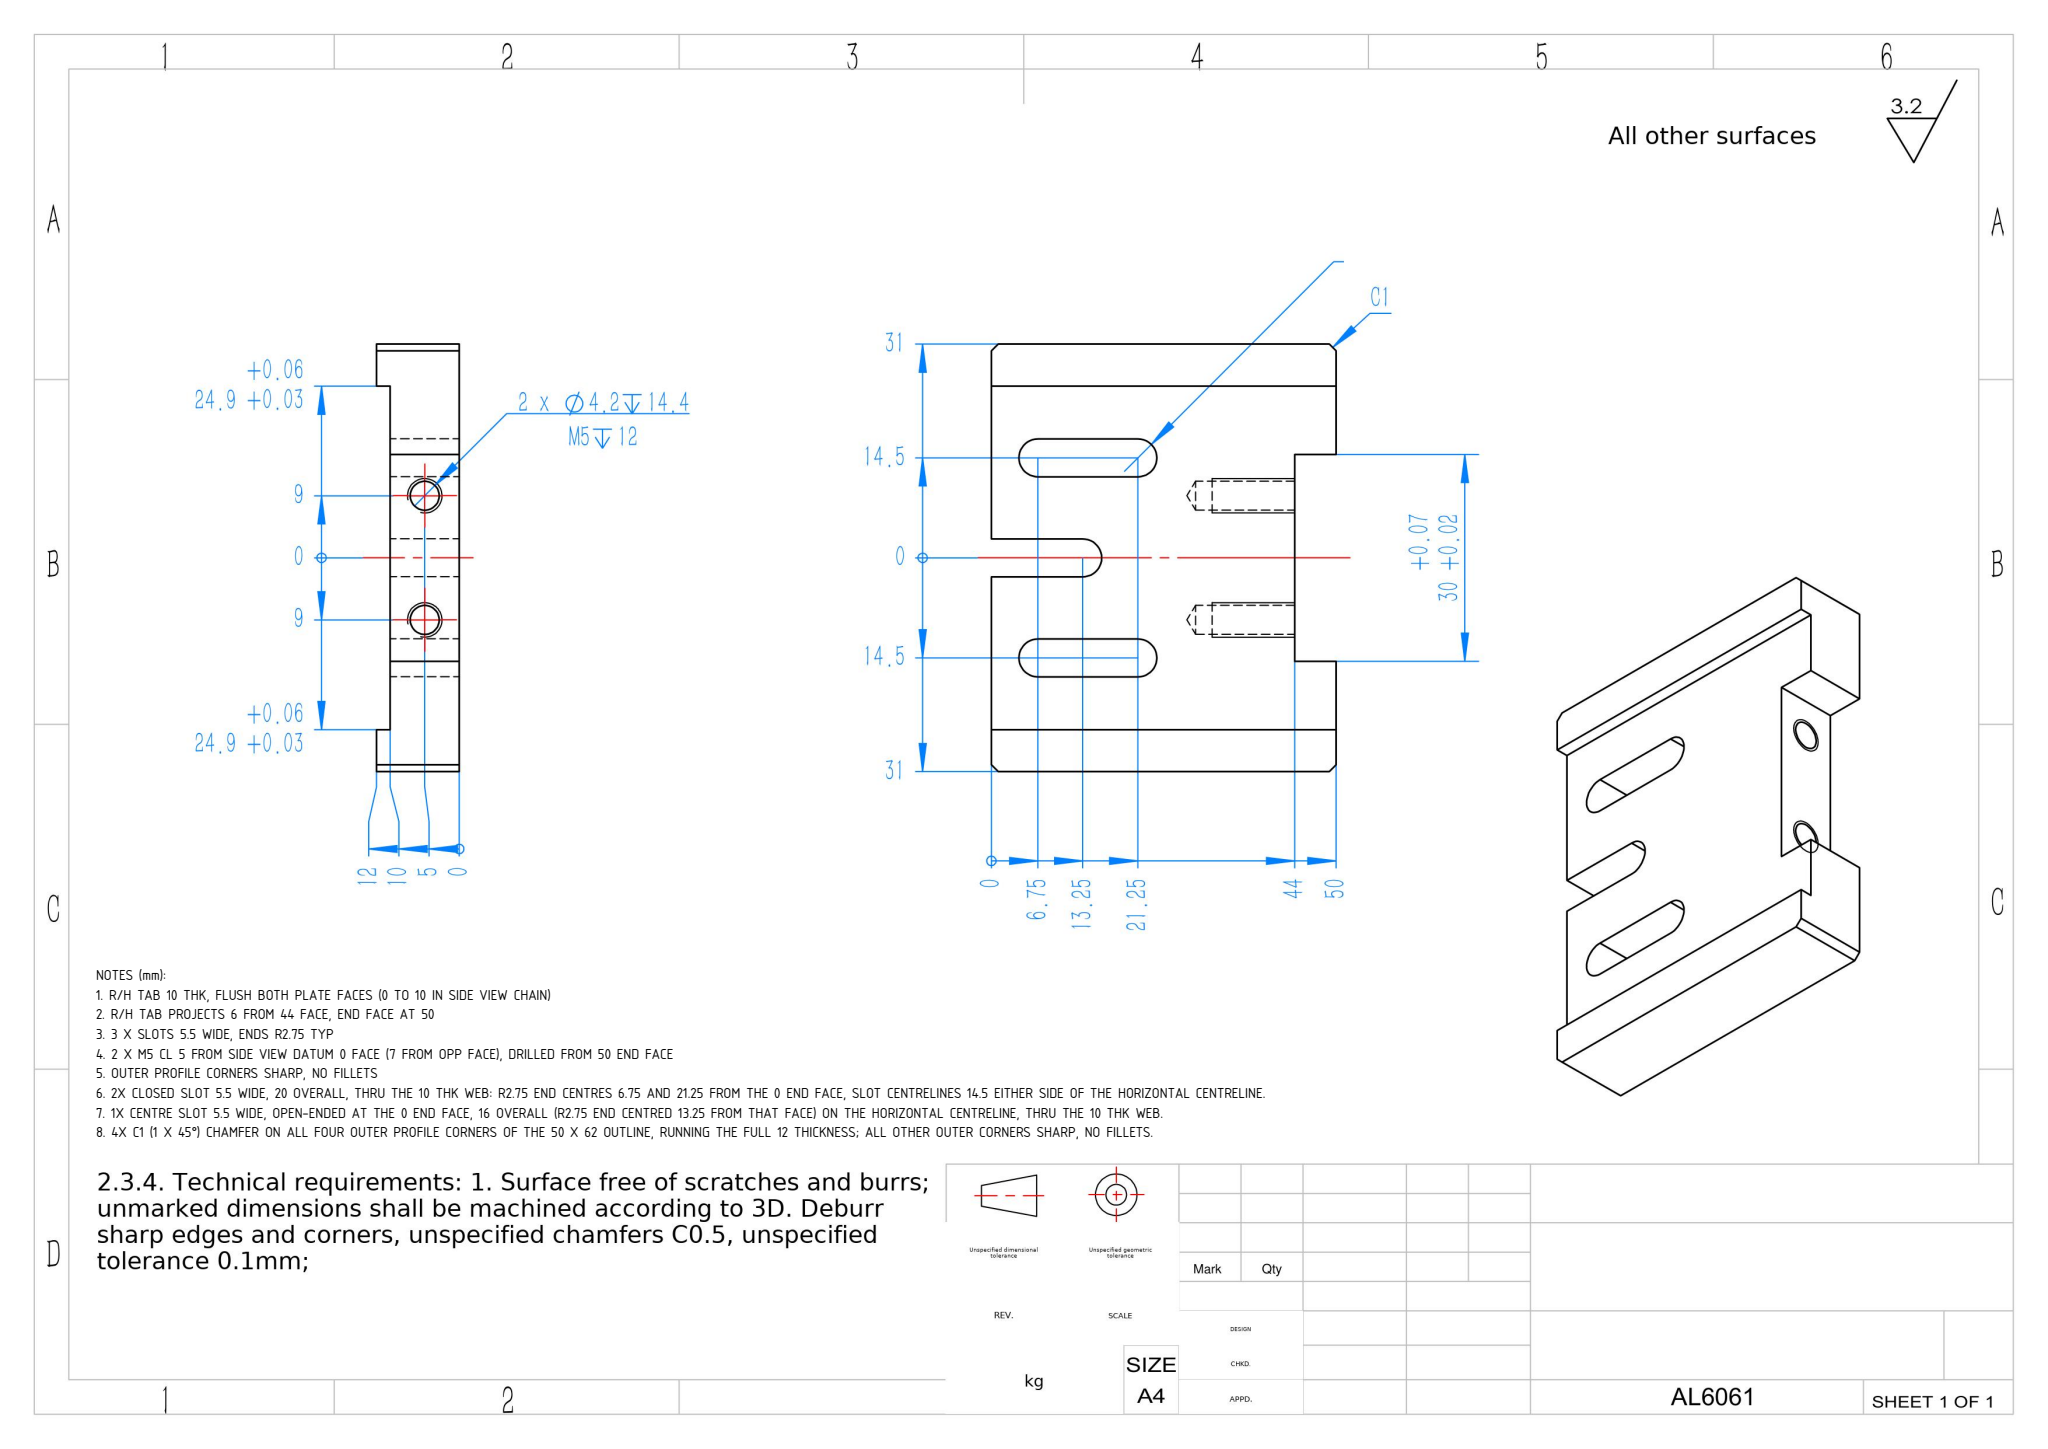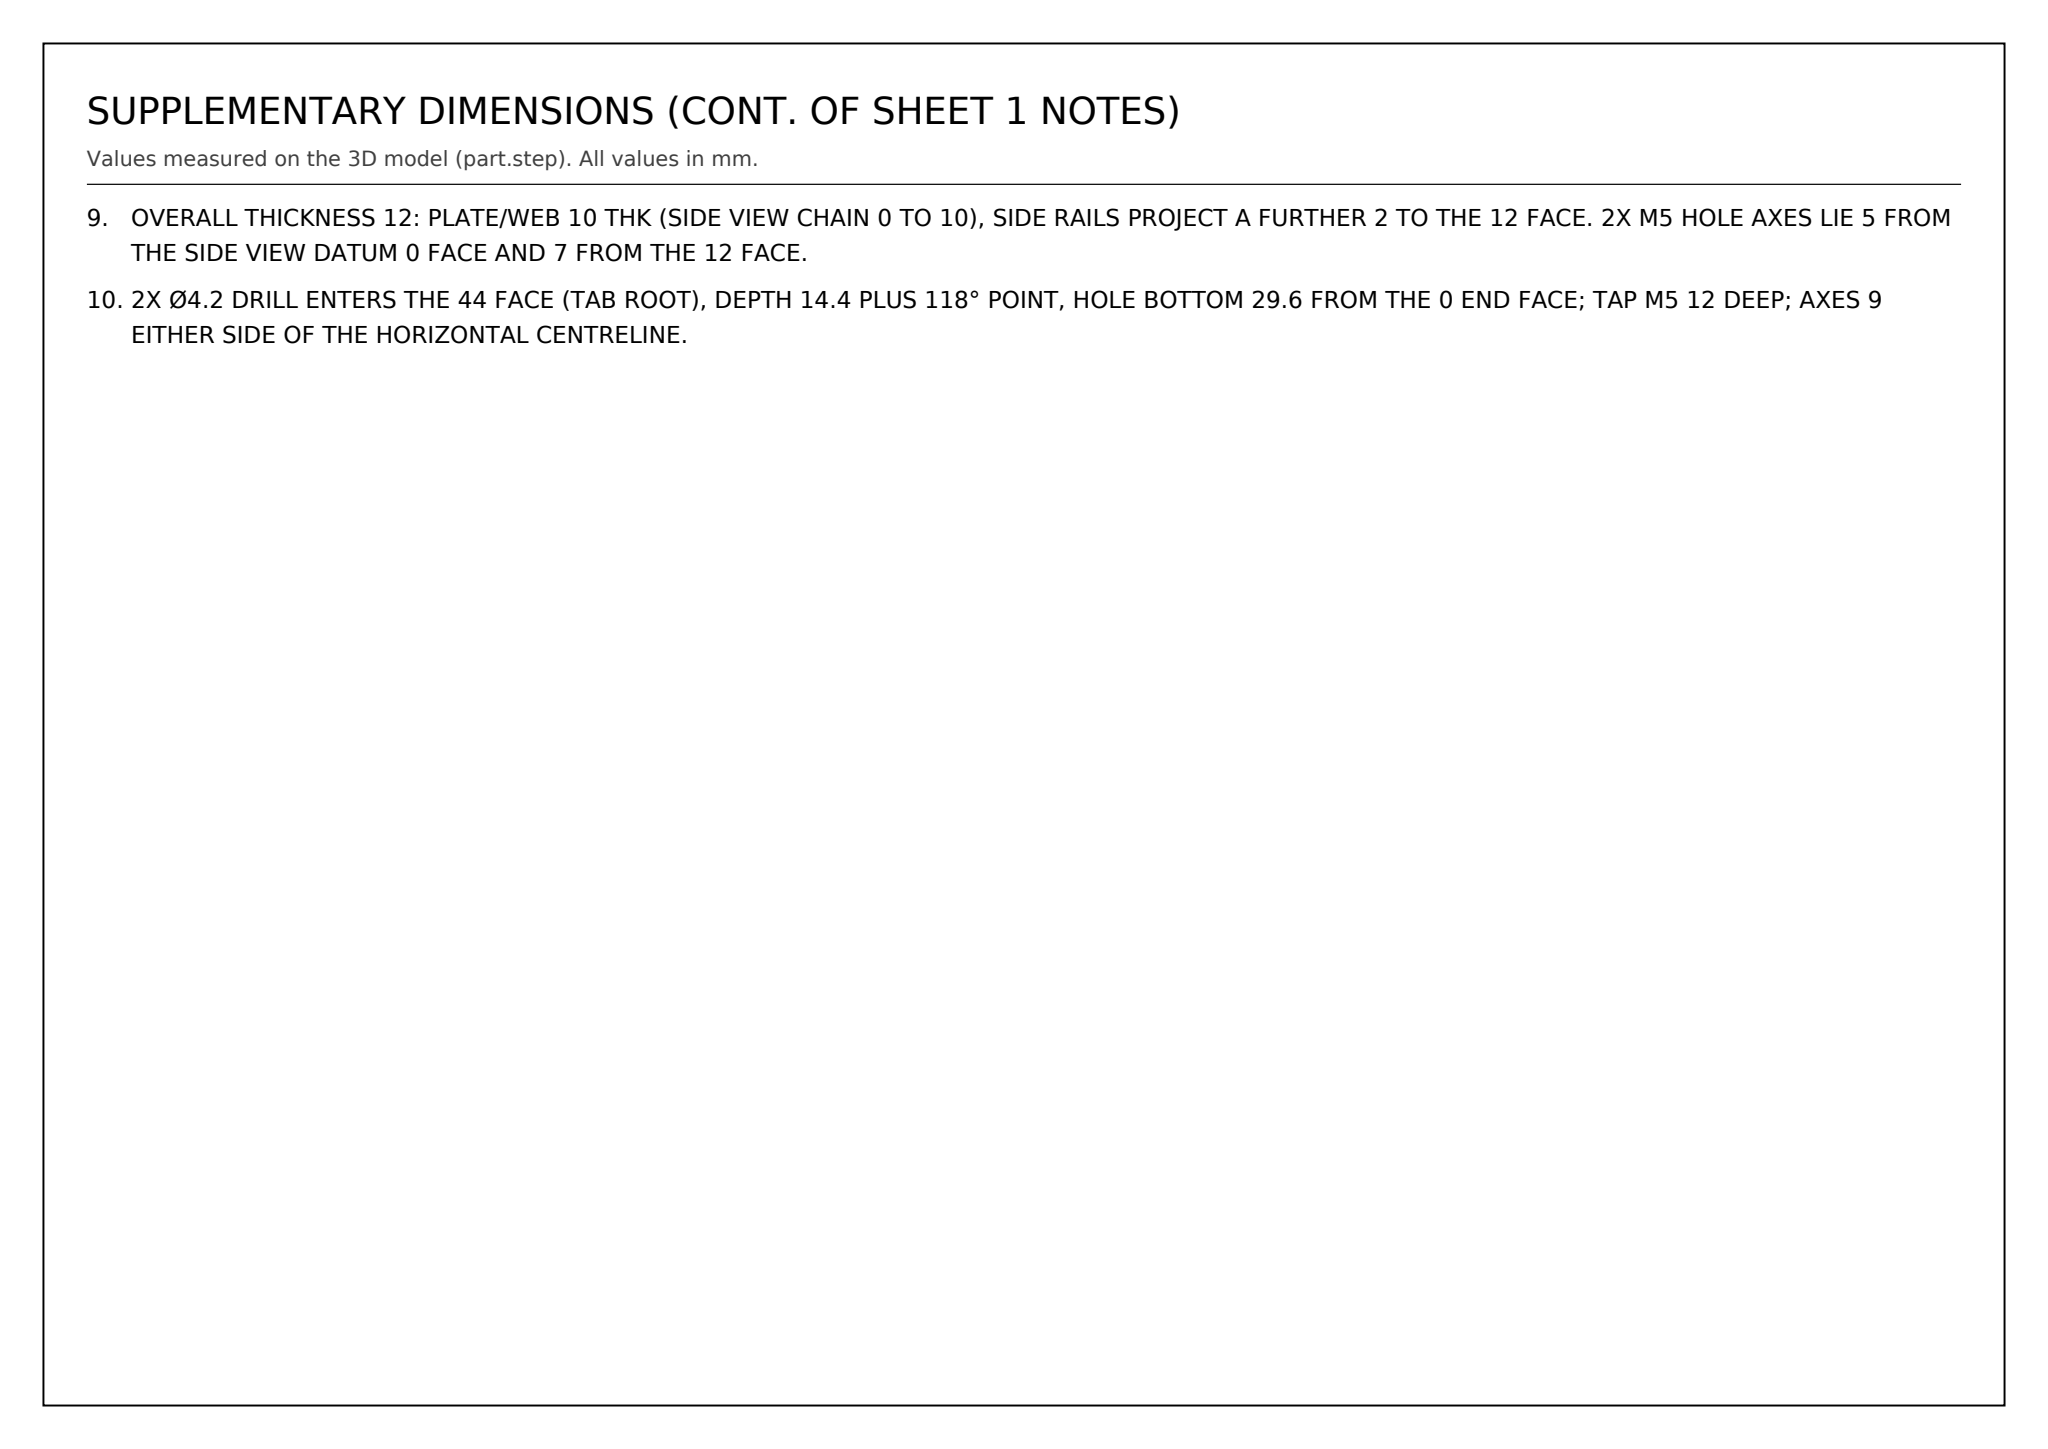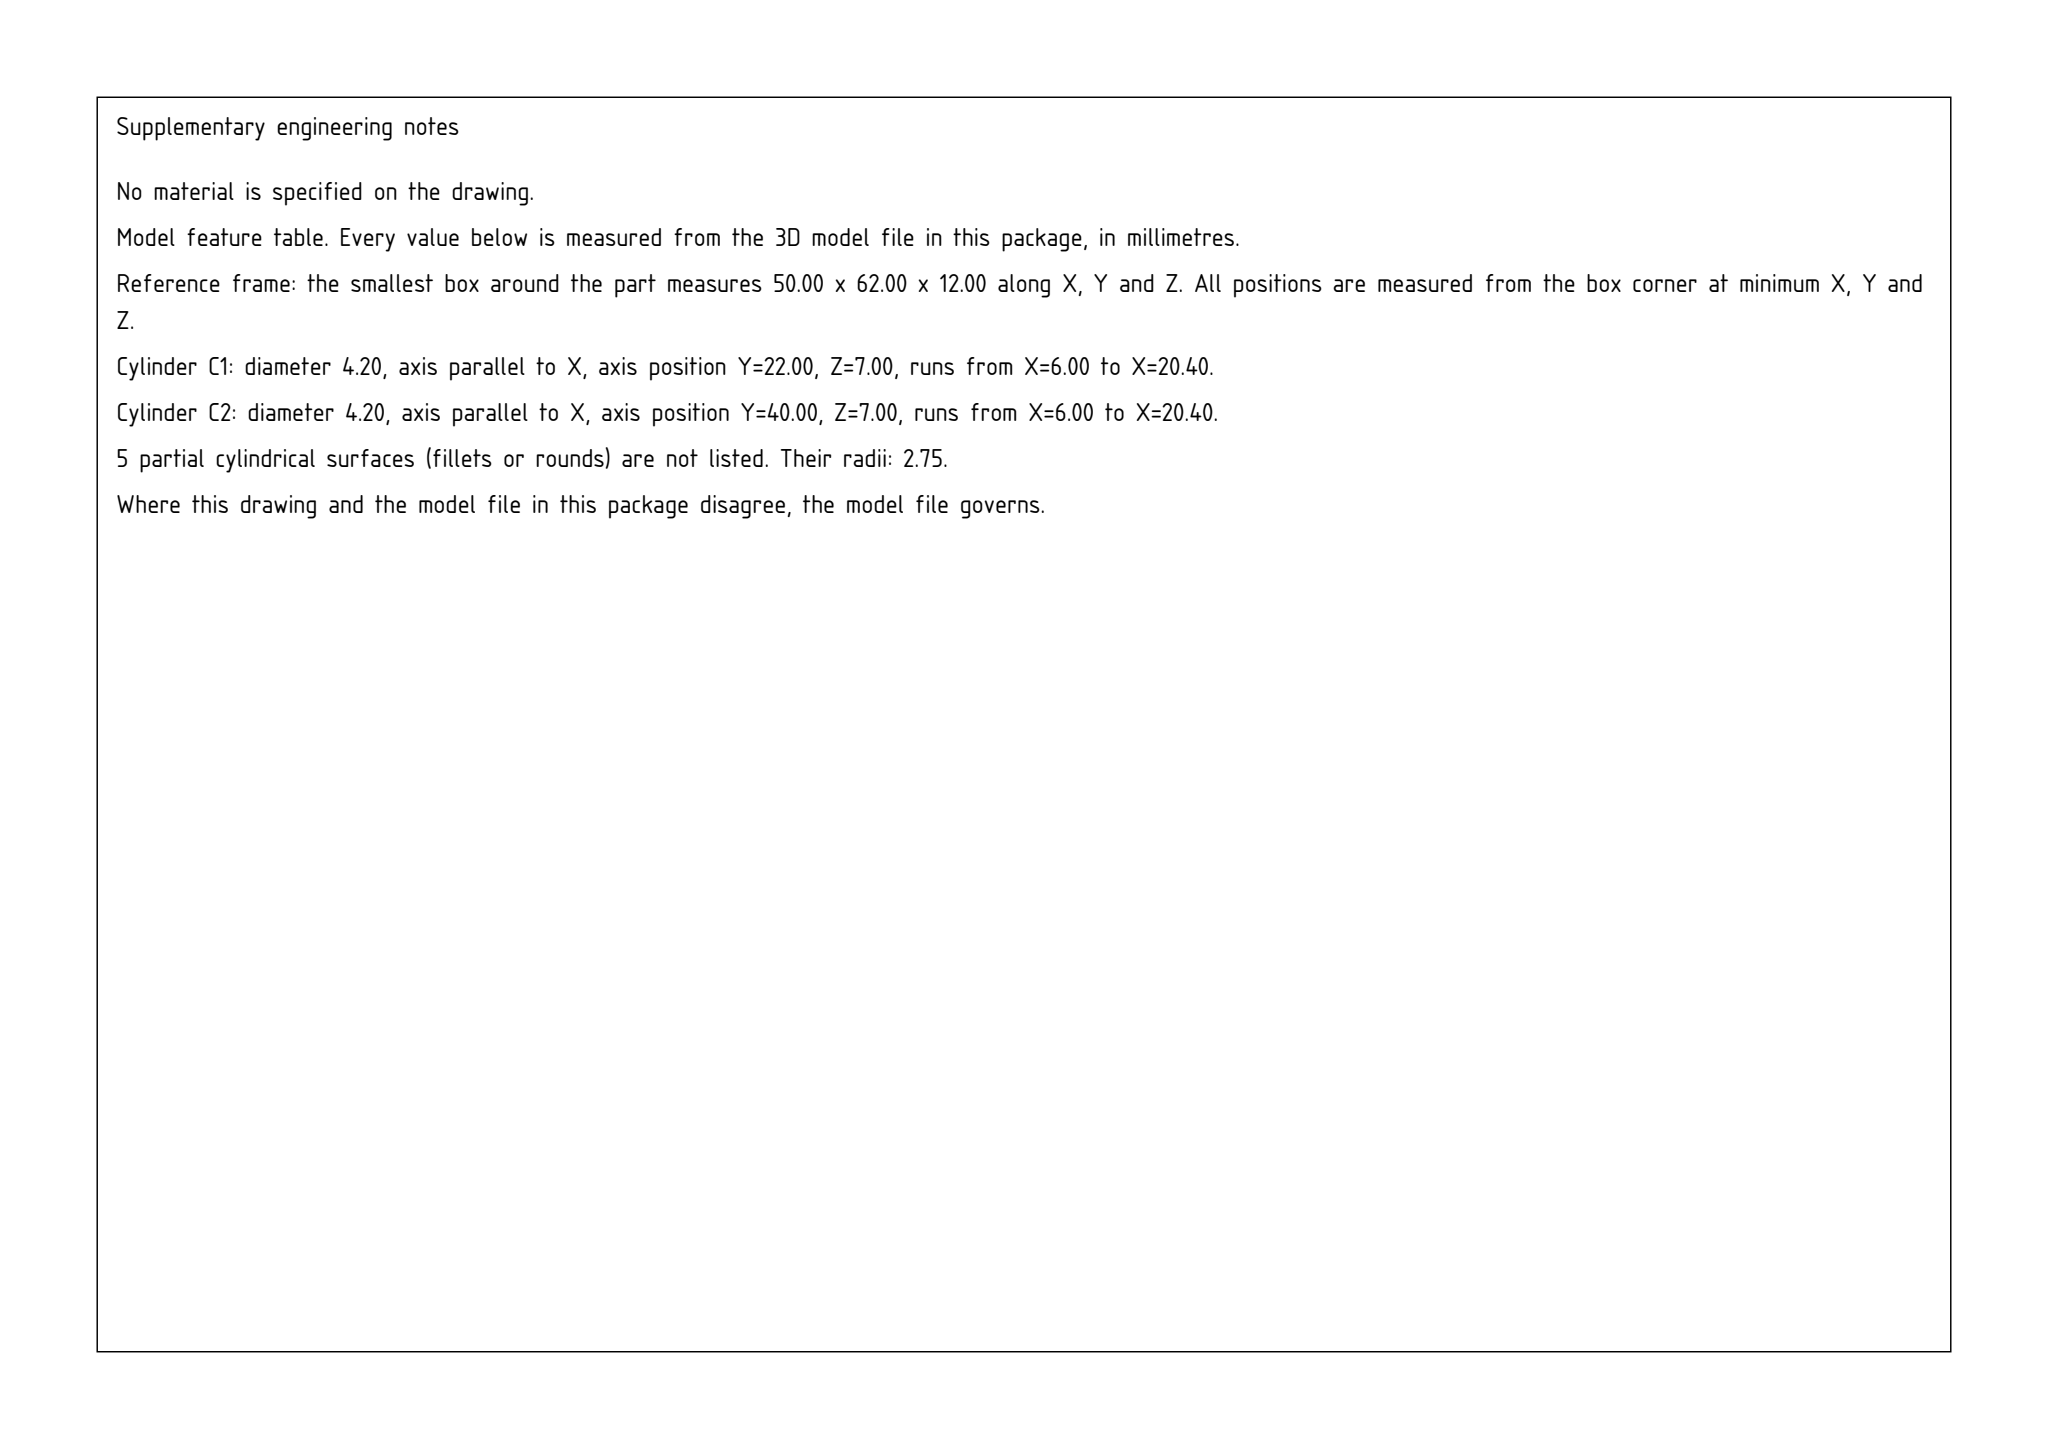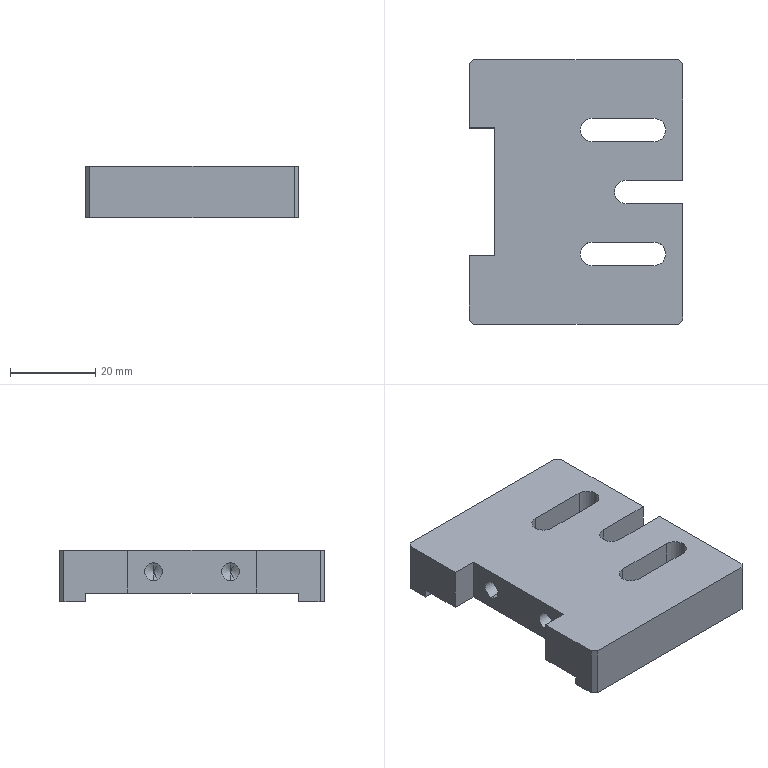Part | SolidWorks | mm | 1 solid | 40 faces | box 50 x 62 x 12 mm | volume 27068 mm3 | plane 25 | cylinder 11 | cone 4 | commonest cylinder face diameters 5.5 x7 4.2 x4
Drawing notes:
R/H TAB 10 THK, FLUSH BOTH PLATE FACES (0 TO 10 IN SIDE VIEW CHAIN) | from the solid: Tab y16-46 (=30) between z-planes 2 and 12 -> 10 thk; side chain 0,5,10,12 from z=12 face
R/H TAB PROJECTS 6 FROM 44 FACE, END FACE AT 50 | from the solid: bbox X=50; x-planes at 0 and 6 -> dwg chain 50 and 44, tab projection 6
3 X SLOTS 5.5 WIDE, ENDS R2.75 TYP | from the solid: cylinders dia 5.5 axis z at (28.75,16.5),(43.25,16.5),(28.75,45.5),(43.25,45.5),(36.75,31.0), len 10
2 X M5 CL 5 FROM SIDE VIEW DATUM 0 FACE (7 FROM OPP FACE), DRILLED FROM 50 END FACE | from the solid: Ø4.2 cyls axis x at (y=22,z=7),(y=40,z=7) L=14.4 from x=0 face (dwg 50); z faces 0 and 12
OUTER PROFILE CORNERS SHARP, NO FILLETS | from the solid: fillet_radii: [] - no fillet faces in STEP; only planar faces + C1 chamfer
2X CLOSED SLOT 5.5 WIDE, 20 OVERALL, THRU THE 10 THK WEB: R2.75 END CENTRES 6.75 AND 21.25 FROM THE 0 END FACE, SLOT CENTRELINES 14.5 EITHER SIDE OF THE HORIZONTAL CENTRELINE. | from the solid: concave arcs D5.5 z-axis at (28.8,16.5),(43.3,16.5),(28.8,45.5),(43.3,45.5), z from 2.0 to 12.0; planes y=13.7/19.2 and y=42.8/48.2 over x 28.8-43.3
1X CENTRE SLOT 5.5 WIDE, OPEN-ENDED AT THE 0 END FACE, 16 OVERALL (R2.75 END CENTRED 13.25 FROM THAT FACE) ON THE HORIZONTAL CENTRELINE, THRU THE 10 THK WEB. | from the solid: concave arc D5.5 z-axis at (36.8,31.0) z 2.0-12.0 with planes y=28.2 and y=33.7 running x 36.8 to 50.0 (open at the x=50 end face)
4X C1 (1 X 45°) CHAMFER ON ALL FOUR OUTER PROFILE CORNERS OF THE 50 X 62 OUTLINE, RUNNING THE FULL 12 THICKNESS; ALL OTHER OUTER CORNERS SHARP, NO FILLETS. | from the solid: inclined_planes: four 45°/45°/90° faces size 1.0 x 1.0 x 12.0 at bbox corners (0,0,0),(0,61,0),(49,0,0),(49,61,0)
OVERALL THICKNESS 12: PLATE/WEB 10 THK (SIDE VIEW CHAIN 0 TO 10), SIDE RAILS PROJECT A FURTHER 2 TO THE 12 FACE. 2X M5 HOLE AXES LIE 5 FROM THE SIDE VIEW DATUM 0 FACE AND 7 FROM THE 12 FACE. | from the solid: bbox_xyz z = 12.0; plane z=12.0 (full face) and plane z=2.0 over x 0-50, y 6.1-55.9 (web underside); planes z=0 only at y 0-6.1 and 55.9-62; holes D4.2 axis x at z = 7.0
2X Ø4.2 DRILL ENTERS THE 44 FACE (TAB ROOT), DEPTH 14.4 PLUS 118° POINT, HOLE BOTTOM 29.6 FROM THE 0 END FACE; TAP M5 12 DEEP; AXES 9 EITHER SIDE OF THE HORIZONTAL CENTRELINE. | from the solid: hole/bore D4.2 axis x from 6.0 to 20.4 at y=22.0 and y=40.0, z=7.0 (bbox x = 50, so entry face is 44 from the x=50 datum end); cones included_angle 118° ref_dia 4.2 at x 20.4-21.7